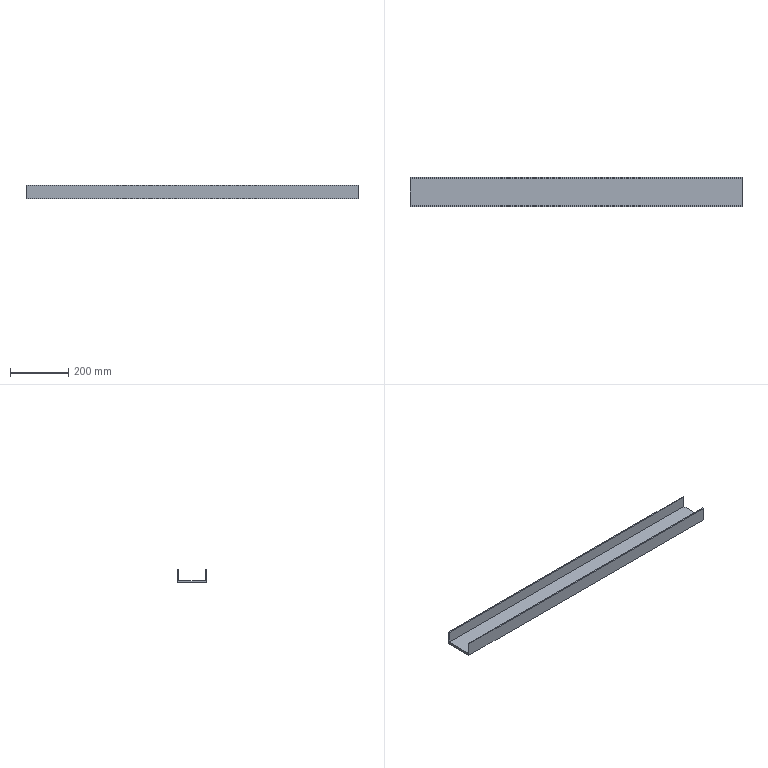Component | SolidWorks | BaseAssembly-1_ChannelSteelAssembly-1_10#ChannelSteel2-2 | 1 solid | 10 faces | box 1140 x 100 x 48 mm | volume 1276800 mm3 | plane 10
build123d program:
from build123d import *

# Parameters (mm, degrees)
EXTRUDE1_DEPTH = 1140


with BuildPart() as part:
    # Sketch1 → Extrude1 (new body)
    with BuildSketch(Plane.XY):
        Polygon((0, 0), (-48, 0), (-48, 100), (0, 100), (0, 96), (-40, 96), (-40, 4), (0, 4), align=None)
    extrude(amount=EXTRUDE1_DEPTH)


solid = part.part

# Placed as in the assembly
solid = solid.moved(Location((722.782, -182.9, 400), (0, -90, 0)))
STEP:
#1=COLOUR_RGB('',0.7922,0.8196,0.9333);
#2=FILL_AREA_STYLE_COLOUR('',#1);
#3=FILL_AREA_STYLE('',(#2));
#4=SURFACE_STYLE_FILL_AREA(#3);
#5=SURFACE_SIDE_STYLE('',(#4));
#6=SURFACE_STYLE_USAGE(.BOTH.,#5);
#7=PRESENTATION_STYLE_ASSIGNMENT((#6));
#8=CARTESIAN_POINT('',(28.456,-7.201,15.748));
#9=VERTEX_POINT('',#8);
#10=CARTESIAN_POINT('',(28.456,-7.043,15.748));
#11=VERTEX_POINT('',#10);
#12=CARTESIAN_POINT('',(28.456,-7.043,15.748));
#13=DIRECTION('',(-0.,1.,0.));
#14=VECTOR('',#13,39.37);
#15=LINE('',#12,#14);
#16=EDGE_CURVE('',#9,#11,#15,.T.);
#17=ORIENTED_EDGE('',*,*,#16,.T.);
#18=CARTESIAN_POINT('',(-16.426,-7.043,15.748));
#19=VERTEX_POINT('',#18);
#20=CARTESIAN_POINT('',(-16.426,-7.043,15.748));
#21=DIRECTION('',(1.,0.,-0.));
#22=VECTOR('',#21,39.37);
#23=LINE('',#20,#22);
#24=EDGE_CURVE('',#19,#11,#23,.T.);
#25=ORIENTED_EDGE('',*,*,#24,.F.);
#26=CARTESIAN_POINT('',(-16.426,-7.201,15.748));
#27=VERTEX_POINT('',#26);
#28=CARTESIAN_POINT('',(-16.426,-7.043,15.748));
#29=DIRECTION('',(-0.,1.,0.));
#30=VECTOR('',#29,39.37);
#31=LINE('',#28,#30);
#32=EDGE_CURVE('',#27,#19,#31,.T.);
#33=ORIENTED_EDGE('',*,*,#32,.F.);
#34=CARTESIAN_POINT('',(-16.426,-7.201,15.748));
#35=DIRECTION('',(1.,0.,-0.));
#36=VECTOR('',#35,39.37);
#37=LINE('',#34,#36);
#38=EDGE_CURVE('',#27,#9,#37,.T.);
#39=ORIENTED_EDGE('',*,*,#38,.T.);
#40=EDGE_LOOP('',(#17,#25,#33,#39));
#41=FACE_OUTER_BOUND('',#40,.T.);
#42=CARTESIAN_POINT('',(-16.426,-7.043,15.748));
#43=DIRECTION('',(-0.,0.,-1.));
#44=DIRECTION('',(0.,-1.,-0.));
#45=AXIS2_PLACEMENT_3D('',#42,#43,#44);
#46=PLANE('',#45);
#47=ADVANCED_FACE('',(#41),#46,.F.);
#48=CARTESIAN_POINT('',(28.456,-7.043,14.173));
#49=VERTEX_POINT('',#48);
#50=CARTESIAN_POINT('',(28.456,-7.043,14.173));
#51=DIRECTION('',(0.,-0.,-1.));
#52=VECTOR('',#51,39.37);
#53=LINE('',#50,#52);
#54=EDGE_CURVE('',#11,#49,#53,.T.);
#55=ORIENTED_EDGE('',*,*,#54,.T.);
#56=CARTESIAN_POINT('',(-16.426,-7.043,14.173));
#57=VERTEX_POINT('',#56);
#58=CARTESIAN_POINT('',(-16.426,-7.043,14.173));
#59=DIRECTION('',(1.,0.,-0.));
#60=VECTOR('',#59,39.37);
#61=LINE('',#58,#60);
#62=EDGE_CURVE('',#57,#49,#61,.T.);
#63=ORIENTED_EDGE('',*,*,#62,.F.);
#64=CARTESIAN_POINT('',(-16.426,-7.043,14.173));
#65=DIRECTION('',(0.,-0.,-1.));
#66=VECTOR('',#65,39.37);
#67=LINE('',#64,#66);
#68=EDGE_CURVE('',#19,#57,#67,.T.);
#69=ORIENTED_EDGE('',*,*,#68,.F.);
#70=ORIENTED_EDGE('',*,*,#24,.T.);
#71=EDGE_LOOP('',(#55,#63,#69,#70));
#72=FACE_OUTER_BOUND('',#71,.T.);
#73=CARTESIAN_POINT('',(-16.426,-7.043,14.173));
#74=DIRECTION('',(0.,-1.,0.));
#75=DIRECTION('',(1.,0.,-0.));
#76=AXIS2_PLACEMENT_3D('',#73,#74,#75);
#77=PLANE('',#76);
#78=ADVANCED_FACE('',(#72),#77,.F.);
#79=CARTESIAN_POINT('',(28.456,-3.421,14.173));
#80=VERTEX_POINT('',#79);
#81=CARTESIAN_POINT('',(28.456,-3.421,14.173));
#82=DIRECTION('',(-0.,1.,-0.));
#83=VECTOR('',#82,39.37);
#84=LINE('',#81,#83);
#85=EDGE_CURVE('',#49,#80,#84,.T.);
#86=ORIENTED_EDGE('',*,*,#85,.T.);
#87=CARTESIAN_POINT('',(-16.426,-3.421,14.173));
#88=VERTEX_POINT('',#87);
#89=CARTESIAN_POINT('',(-16.426,-3.421,14.173));
#90=DIRECTION('',(1.,0.,-0.));
#91=VECTOR('',#90,39.37);
#92=LINE('',#89,#91);
#93=EDGE_CURVE('',#88,#80,#92,.T.);
#94=ORIENTED_EDGE('',*,*,#93,.F.);
#95=CARTESIAN_POINT('',(-16.426,-3.421,14.173));
#96=DIRECTION('',(-0.,1.,-0.));
#97=VECTOR('',#96,39.37);
#98=LINE('',#95,#97);
#99=EDGE_CURVE('',#57,#88,#98,.T.);
#100=ORIENTED_EDGE('',*,*,#99,.F.);
#101=ORIENTED_EDGE('',*,*,#62,.T.);
#102=EDGE_LOOP('',(#86,#94,#100,#101));
#103=FACE_OUTER_BOUND('',#102,.T.);
#104=CARTESIAN_POINT('',(-16.426,-3.421,14.173));
#105=DIRECTION('',(0.,-0.,-1.));
#106=DIRECTION('',(0.,-1.,0.));
#107=AXIS2_PLACEMENT_3D('',#104,#105,#106);
#108=PLANE('',#107);
#109=ADVANCED_FACE('',(#103),#108,.F.);
#110=CARTESIAN_POINT('',(28.456,-3.421,15.748));
#111=VERTEX_POINT('',#110);
#112=CARTESIAN_POINT('',(28.456,-3.421,15.748));
#113=DIRECTION('',(0.,0.,1.));
#114=VECTOR('',#113,39.37);
#115=LINE('',#112,#114);
#116=EDGE_CURVE('',#80,#111,#115,.T.);
#117=ORIENTED_EDGE('',*,*,#116,.T.);
#118=CARTESIAN_POINT('',(-16.426,-3.421,15.748));
#119=VERTEX_POINT('',#118);
#120=CARTESIAN_POINT('',(-16.426,-3.421,15.748));
#121=DIRECTION('',(1.,0.,-0.));
#122=VECTOR('',#121,39.37);
#123=LINE('',#120,#122);
#124=EDGE_CURVE('',#119,#111,#123,.T.);
#125=ORIENTED_EDGE('',*,*,#124,.F.);
#126=CARTESIAN_POINT('',(-16.426,-3.421,15.748));
#127=DIRECTION('',(0.,0.,1.));
#128=VECTOR('',#127,39.37);
#129=LINE('',#126,#128);
#130=EDGE_CURVE('',#88,#119,#129,.T.);
#131=ORIENTED_EDGE('',*,*,#130,.F.);
#132=ORIENTED_EDGE('',*,*,#93,.T.);
#133=EDGE_LOOP('',(#117,#125,#131,#132));
#134=FACE_OUTER_BOUND('',#133,.T.);
#135=CARTESIAN_POINT('',(-16.426,-3.421,15.748));
#136=DIRECTION('',(-0.,1.,-0.));
#137=DIRECTION('',(-1.,-0.,0.));
#138=AXIS2_PLACEMENT_3D('',#135,#136,#137);
#139=PLANE('',#138);
#140=ADVANCED_FACE('',(#134),#139,.F.);
#141=CARTESIAN_POINT('',(28.456,-3.264,15.748));
#142=VERTEX_POINT('',#141);
#143=CARTESIAN_POINT('',(28.456,-3.264,15.748));
#144=DIRECTION('',(-0.,1.,-0.));
#145=VECTOR('',#144,39.37);
#146=LINE('',#143,#145);
#147=EDGE_CURVE('',#111,#142,#146,.T.);
#148=ORIENTED_EDGE('',*,*,#147,.T.);
#149=CARTESIAN_POINT('',(-16.426,-3.264,15.748));
#150=VERTEX_POINT('',#149);
#151=CARTESIAN_POINT('',(-16.426,-3.264,15.748));
#152=DIRECTION('',(1.,0.,-0.));
#153=VECTOR('',#152,39.37);
#154=LINE('',#151,#153);
#155=EDGE_CURVE('',#150,#142,#154,.T.);
#156=ORIENTED_EDGE('',*,*,#155,.F.);
#157=CARTESIAN_POINT('',(-16.426,-3.264,15.748));
#158=DIRECTION('',(-0.,1.,-0.));
#159=VECTOR('',#158,39.37);
#160=LINE('',#157,#159);
#161=EDGE_CURVE('',#119,#150,#160,.T.);
#162=ORIENTED_EDGE('',*,*,#161,.F.);
#163=ORIENTED_EDGE('',*,*,#124,.T.);
#164=EDGE_LOOP('',(#148,#156,#162,#163));
#165=FACE_OUTER_BOUND('',#164,.T.);
#166=CARTESIAN_POINT('',(-16.426,-3.264,15.748));
#167=DIRECTION('',(0.,-0.,-1.));
#168=DIRECTION('',(-1.,-0.,0.));
#169=AXIS2_PLACEMENT_3D('',#166,#167,#168);
#170=PLANE('',#169);
#171=ADVANCED_FACE('',(#165),#170,.F.);
#172=CARTESIAN_POINT('',(28.456,-3.264,13.858));
#173=VERTEX_POINT('',#172);
#174=CARTESIAN_POINT('',(28.456,-3.264,13.858));
#175=DIRECTION('',(0.,-0.,-1.));
#176=VECTOR('',#175,39.37);
#177=LINE('',#174,#176);
#178=EDGE_CURVE('',#142,#173,#177,.T.);
#179=ORIENTED_EDGE('',*,*,#178,.T.);
#180=CARTESIAN_POINT('',(-16.426,-3.264,13.858));
#181=VERTEX_POINT('',#180);
#182=CARTESIAN_POINT('',(-16.426,-3.264,13.858));
#183=DIRECTION('',(1.,0.,-0.));
#184=VECTOR('',#183,39.37);
#185=LINE('',#182,#184);
#186=EDGE_CURVE('',#181,#173,#185,.T.);
#187=ORIENTED_EDGE('',*,*,#186,.F.);
#188=CARTESIAN_POINT('',(-16.426,-3.264,13.858));
#189=DIRECTION('',(0.,-0.,-1.));
#190=VECTOR('',#189,39.37);
#191=LINE('',#188,#190);
#192=EDGE_CURVE('',#150,#181,#191,.T.);
#193=ORIENTED_EDGE('',*,*,#192,.F.);
#194=ORIENTED_EDGE('',*,*,#155,.T.);
#195=EDGE_LOOP('',(#179,#187,#193,#194));
#196=FACE_OUTER_BOUND('',#195,.T.);
#197=CARTESIAN_POINT('',(-16.426,-3.264,13.858));
#198=DIRECTION('',(0.,-1.,0.));
#199=DIRECTION('',(1.,0.,-0.));
#200=AXIS2_PLACEMENT_3D('',#197,#198,#199);
#201=PLANE('',#200);
#202=ADVANCED_FACE('',(#196),#201,.F.);
#203=CARTESIAN_POINT('',(28.456,-7.201,13.858));
#204=VERTEX_POINT('',#203);
#205=CARTESIAN_POINT('',(28.456,-7.201,13.858));
#206=DIRECTION('',(0.,-1.,0.));
#207=VECTOR('',#206,39.37);
#208=LINE('',#205,#207);
#209=EDGE_CURVE('',#173,#204,#208,.T.);
#210=ORIENTED_EDGE('',*,*,#209,.T.);
#211=CARTESIAN_POINT('',(-16.426,-7.201,13.858));
#212=VERTEX_POINT('',#211);
#213=CARTESIAN_POINT('',(-16.426,-7.201,13.858));
#214=DIRECTION('',(1.,0.,-0.));
#215=VECTOR('',#214,39.37);
#216=LINE('',#213,#215);
#217=EDGE_CURVE('',#212,#204,#216,.T.);
#218=ORIENTED_EDGE('',*,*,#217,.F.);
#219=CARTESIAN_POINT('',(-16.426,-7.201,13.858));
#220=DIRECTION('',(0.,-1.,0.));
#221=VECTOR('',#220,39.37);
#222=LINE('',#219,#221);
#223=EDGE_CURVE('',#181,#212,#222,.T.);
#224=ORIENTED_EDGE('',*,*,#223,.F.);
#225=ORIENTED_EDGE('',*,*,#186,.T.);
#226=EDGE_LOOP('',(#210,#218,#224,#225));
#227=FACE_OUTER_BOUND('',#226,.T.);
#228=CARTESIAN_POINT('',(-16.426,-7.201,13.858));
#229=DIRECTION('',(0.,0.,1.));
#230=DIRECTION('',(1.,0.,-0.));
#231=AXIS2_PLACEMENT_3D('',#228,#229,#230);
#232=PLANE('',#231);
#233=ADVANCED_FACE('',(#227),#232,.F.);
#234=CARTESIAN_POINT('',(28.456,-7.201,15.748));
#235=DIRECTION('',(-0.,0.,1.));
#236=VECTOR('',#235,39.37);
#237=LINE('',#234,#236);
#238=EDGE_CURVE('',#204,#9,#237,.T.);
#239=ORIENTED_EDGE('',*,*,#238,.T.);
#240=ORIENTED_EDGE('',*,*,#38,.F.);
#241=CARTESIAN_POINT('',(-16.426,-7.201,15.748));
#242=DIRECTION('',(-0.,0.,1.));
#243=VECTOR('',#242,39.37);
#244=LINE('',#241,#243);
#245=EDGE_CURVE('',#212,#27,#244,.T.);
#246=ORIENTED_EDGE('',*,*,#245,.F.);
#247=ORIENTED_EDGE('',*,*,#217,.T.);
#248=EDGE_LOOP('',(#239,#240,#246,#247));
#249=FACE_OUTER_BOUND('',#248,.T.);
#250=CARTESIAN_POINT('',(-16.426,-7.201,15.748));
#251=DIRECTION('',(-0.,1.,-0.));
#252=DIRECTION('',(0.,-0.,-1.));
#253=AXIS2_PLACEMENT_3D('',#250,#251,#252);
#254=PLANE('',#253);
#255=ADVANCED_FACE('',(#249),#254,.F.);
#256=ORIENTED_EDGE('',*,*,#32,.T.);
#257=ORIENTED_EDGE('',*,*,#68,.T.);
#258=ORIENTED_EDGE('',*,*,#99,.T.);
#259=ORIENTED_EDGE('',*,*,#130,.T.);
#260=ORIENTED_EDGE('',*,*,#161,.T.);
#261=ORIENTED_EDGE('',*,*,#192,.T.);
#262=ORIENTED_EDGE('',*,*,#223,.T.);
#263=ORIENTED_EDGE('',*,*,#245,.T.);
#264=EDGE_LOOP('',(#256,#257,#258,#259,#260,#261,#262,#263));
#265=FACE_OUTER_BOUND('',#264,.T.);
#266=CARTESIAN_POINT('',(-16.426,-3.264,15.748));
#267=DIRECTION('',(-1.,-0.,0.));
#268=DIRECTION('',(0.,0.,1.));
#269=AXIS2_PLACEMENT_3D('',#266,#267,#268);
#270=PLANE('',#269);
#271=ADVANCED_FACE('',(#265),#270,.T.);
#272=ORIENTED_EDGE('',*,*,#16,.F.);
#273=ORIENTED_EDGE('',*,*,#238,.F.);
#274=ORIENTED_EDGE('',*,*,#209,.F.);
#275=ORIENTED_EDGE('',*,*,#178,.F.);
#276=ORIENTED_EDGE('',*,*,#147,.F.);
#277=ORIENTED_EDGE('',*,*,#116,.F.);
#278=ORIENTED_EDGE('',*,*,#85,.F.);
#279=ORIENTED_EDGE('',*,*,#54,.F.);
#280=EDGE_LOOP('',(#272,#273,#274,#275,#276,#277,#278,#279));
#281=FACE_OUTER_BOUND('',#280,.T.);
#282=CARTESIAN_POINT('',(28.456,-3.264,15.748));
#283=DIRECTION('',(-1.,-0.,0.));
#284=DIRECTION('',(0.,0.,1.));
#285=AXIS2_PLACEMENT_3D('',#282,#283,#284);
#286=PLANE('',#285);
#287=ADVANCED_FACE('',(#281),#286,.F.);
#288=CLOSED_SHELL('',(#47,#78,#109,#140,#171,#202,#233,#255,#271,#287));
#289=MANIFOLD_SOLID_BREP('',#288);
#290=STYLED_ITEM('',(#7),#289);
#291=PRESENTATION_LAYER_ASSIGNMENT('','',(#290));
#292=(LENGTH_UNIT()NAMED_UNIT(*)SI_UNIT($,.METRE.));
#293=LENGTH_MEASURE_WITH_UNIT(LENGTH_MEASURE(0.0254),#292);
#294=DIMENSIONAL_EXPONENTS(1.,0.,0.,0.,0.,0.,0.);
#295=(CONVERSION_BASED_UNIT('',#293)LENGTH_UNIT()NAMED_UNIT(#294));
#296=UNCERTAINTY_MEASURE_WITH_UNIT(LENGTH_MEASURE(0.00001),#295,'','');
#297=(NAMED_UNIT(*)PLANE_ANGLE_UNIT()SI_UNIT($,.RADIAN.));
#298=(NAMED_UNIT(*)SI_UNIT($,.STERADIAN.)SOLID_ANGLE_UNIT());
#299=(GEOMETRIC_REPRESENTATION_CONTEXT(3)GLOBAL_UNCERTAINTY_ASSIGNED_CONTEXT((#296))GLOBAL_UNIT_ASSIGNED_CONTEXT((#295,#297,#298))REPRESENTATION_CONTEXT('',''));
#300=MECHANICAL_DESIGN_GEOMETRIC_PRESENTATION_REPRESENTATION('',(#290),#299);
#301=CARTESIAN_POINT('',(0.,0.,0.));
#302=DIRECTION('',(0.,0.,1.));
#303=DIRECTION('',(1.,0.,0.));
#304=AXIS2_PLACEMENT_3D('',#301,#302,#303);
#305=(LENGTH_UNIT()NAMED_UNIT(*)SI_UNIT($,.METRE.));
#306=LENGTH_MEASURE_WITH_UNIT(LENGTH_MEASURE(0.0254),#305);
#307=DIMENSIONAL_EXPONENTS(1.,0.,0.,0.,0.,0.,0.);
#308=(CONVERSION_BASED_UNIT('',#306)LENGTH_UNIT()NAMED_UNIT(#307));
#309=UNCERTAINTY_MEASURE_WITH_UNIT(LENGTH_MEASURE(0.00001),#308,'','');
#310=(NAMED_UNIT(*)PLANE_ANGLE_UNIT()SI_UNIT($,.RADIAN.));
#311=(NAMED_UNIT(*)SI_UNIT($,.STERADIAN.)SOLID_ANGLE_UNIT());
#312=(GEOMETRIC_REPRESENTATION_CONTEXT(3)GLOBAL_UNCERTAINTY_ASSIGNED_CONTEXT((#309))GLOBAL_UNIT_ASSIGNED_CONTEXT((#308,#310,#311))REPRESENTATION_CONTEXT('',''));
#313=ADVANCED_BREP_SHAPE_REPRESENTATION('',(#289,#304),#312);